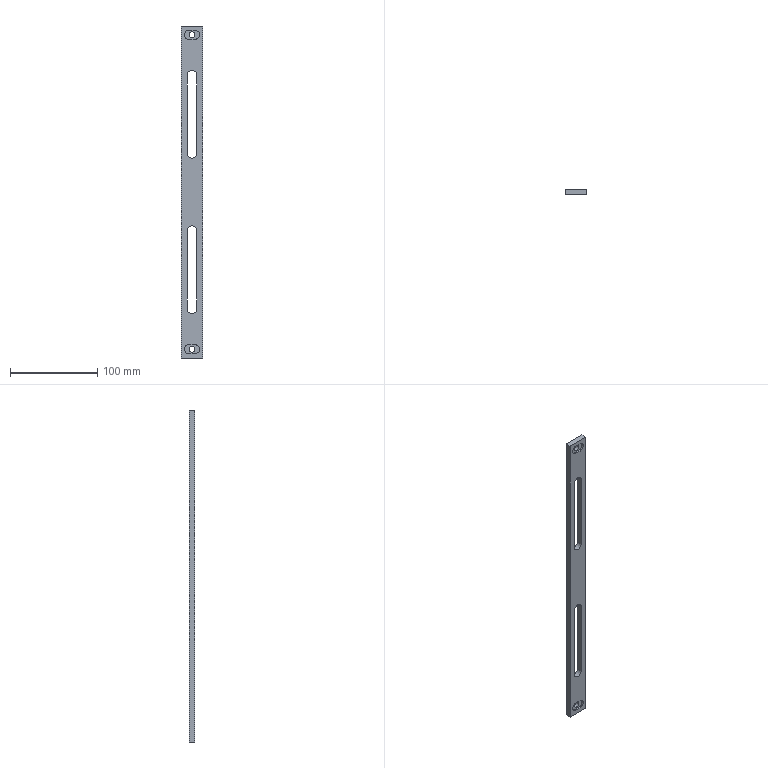Component | SolidWorks | SL021-102-4098.SL4PRT-6 | 1 solid | 30 faces | box 25 x 6 x 380 mm | volume 43743 mm3 | plane 16 | cylinder 14 | commonest cylinder face diameters 10.2 x6 6.5 x4 10.5 x4 | material AL6061
build123d program:
from build123d import *

# Parameters (mm, degrees)
SKETCH1_W                  = 380
SKETCH1_H                  = 25
BOSS_EXTRUDE1_DEPTH        = 3
CUT_EXTRUDE1_DEPTH         = 191.505
F_8_5_8_5_DIAMETER_HOLE1_D = 6.5
CUT_EXTRUDE2_DEPTH         = 2


with BuildPart() as part:
    # Sketch1 → Boss-Extrude1 (new, symmetric)
    with BuildSketch(Plane(origin=(0, 0, 0), x_dir=(1, 0, 0), z_dir=(0, 1, 0))):
        Rectangle(SKETCH1_W, SKETCH1_H)
    extrude(amount=BOSS_EXTRUDE1_DEPTH, both=True)

    # Sketch2 → Cut-Extrude1 (cut, through all)
    with BuildSketch(Plane(origin=(0, 3, 0), x_dir=(1, 0, 0), z_dir=(0, 1, 0))):
        with BuildLine():
            Line((-44, -5.25), (-134, -5.25))
            ThreePointArc((-134, -5.25), (-139.25, 0), (-134, 5.25))
            Line((-134, 5.25), (-44, 5.25))
            ThreePointArc((-44, 5.25), (-38.75, 0), (-44, -5.25))
        make_face()
        with BuildLine():
            Line((44, -5.25), (134, -5.25))
            ThreePointArc((134, -5.25), (139.25, 0), (134, 5.25))
            Line((134, 5.25), (44, 5.25))
            ThreePointArc((44, 5.25), (38.75, 0), (44, -5.25))
        make_face()
    extrude(amount=-CUT_EXTRUDE1_DEPTH, mode=Mode.SUBTRACT)

    # 8.5 _8.5_ Diameter Hole1 (through all)
    with Locations(Plane(origin=(0, -3, 0), x_dir=(-1, 0, 0), z_dir=(0, -1, 0))):
        with Locations((180, 0), (-180, 0)):
            Hole(F_8_5_8_5_DIAMETER_HOLE1_D / 2)

    # Sketch6 → Cut-Extrude2 (cut)
    with BuildSketch(Plane.XZ.offset(3)):
        with BuildLine():
            Line((-174.9, 3.5), (-174.9, -3.5))
            ThreePointArc((-174.9, -3.5), (-180, -8.6), (-185.1, -3.5))
            Line((-185.1, -3.5), (-185.1, 3.5))
            ThreePointArc((-185.1, 3.5), (-180, 8.6), (-174.9, 3.5))
        make_face()
        with BuildLine():
            Line((174.9, 3.5), (174.9, -3.5))
            ThreePointArc((174.9, -3.5), (180, -8.6), (185.1, -3.5))
            Line((185.1, -3.5), (185.1, 3.5))
            ThreePointArc((185.1, 3.5), (180, 8.6), (174.9, 3.5))
        make_face()
    extrude(amount=-CUT_EXTRUDE2_DEPTH, mode=Mode.SUBTRACT)


solid = part.part

# Placed as in the assembly
solid = solid.moved(Location((-48.663, -105.499, -151.378), (0, 90, 0)))
STEP:
#1=COLOUR_RGB('',0.7922,0.8196,0.9333);
#2=FILL_AREA_STYLE_COLOUR('',#1);
#3=FILL_AREA_STYLE('',(#2));
#4=SURFACE_STYLE_FILL_AREA(#3);
#5=SURFACE_SIDE_STYLE('',(#4));
#6=SURFACE_STYLE_USAGE(.BOTH.,#5);
#7=PRESENTATION_STYLE_ASSIGNMENT((#6));
#8=CARTESIAN_POINT('',(-1.577,-4.193,1.127));
#9=VERTEX_POINT('',#8);
#10=CARTESIAN_POINT('',(-1.778,-4.193,1.328));
#11=VERTEX_POINT('',#10);
#12=CARTESIAN_POINT('',(-1.778,-4.193,1.127));
#13=DIRECTION('',(0.,-1.,0.));
#14=DIRECTION('',(-1.,0.,0.));
#15=AXIS2_PLACEMENT_3D('',#12,#13,#14);
#16=CIRCLE('',#15,0.2008);
#17=EDGE_CURVE('',#9,#11,#16,.T.);
#18=ORIENTED_EDGE('',*,*,#17,.F.);
#19=CARTESIAN_POINT('',(-1.577,-4.272,1.127));
#20=VERTEX_POINT('',#19);
#21=CARTESIAN_POINT('',(-1.577,-4.193,1.127));
#22=DIRECTION('',(0.,-1.,0.));
#23=VECTOR('',#22,39.37);
#24=LINE('',#21,#23);
#25=EDGE_CURVE('',#9,#20,#24,.T.);
#26=ORIENTED_EDGE('',*,*,#25,.T.);
#27=CARTESIAN_POINT('',(-1.778,-4.272,1.328));
#28=VERTEX_POINT('',#27);
#29=CARTESIAN_POINT('',(-1.778,-4.272,1.127));
#30=DIRECTION('',(0.,-1.,0.));
#31=DIRECTION('',(-1.,0.,0.));
#32=AXIS2_PLACEMENT_3D('',#29,#30,#31);
#33=CIRCLE('',#32,0.2008);
#34=EDGE_CURVE('',#20,#28,#33,.T.);
#35=ORIENTED_EDGE('',*,*,#34,.T.);
#36=CARTESIAN_POINT('',(-1.778,-4.193,1.328));
#37=DIRECTION('',(0.,-1.,0.));
#38=VECTOR('',#37,39.37);
#39=LINE('',#36,#38);
#40=EDGE_CURVE('',#11,#28,#39,.T.);
#41=ORIENTED_EDGE('',*,*,#40,.F.);
#42=EDGE_LOOP('',(#18,#26,#35,#41));
#43=FACE_OUTER_BOUND('',#42,.T.);
#44=CARTESIAN_POINT('',(-1.778,-4.193,1.127));
#45=DIRECTION('',(0.,-1.,0.));
#46=DIRECTION('',(1.,0.,0.));
#47=AXIS2_PLACEMENT_3D('',#44,#45,#46);
#48=CYLINDRICAL_SURFACE('',#47,0.2008);
#49=ADVANCED_FACE('',(#43),#48,.F.);
#50=CARTESIAN_POINT('',(-1.577,-4.193,-13.046));
#51=VERTEX_POINT('',#50);
#52=CARTESIAN_POINT('',(-1.778,-4.193,-12.846));
#53=VERTEX_POINT('',#52);
#54=CARTESIAN_POINT('',(-1.778,-4.193,-13.046));
#55=DIRECTION('',(0.,-1.,0.));
#56=DIRECTION('',(1.,0.,0.));
#57=AXIS2_PLACEMENT_3D('',#54,#55,#56);
#58=CIRCLE('',#57,0.2008);
#59=EDGE_CURVE('',#51,#53,#58,.T.);
#60=ORIENTED_EDGE('',*,*,#59,.F.);
#61=CARTESIAN_POINT('',(-1.577,-4.272,-13.046));
#62=VERTEX_POINT('',#61);
#63=CARTESIAN_POINT('',(-1.577,-4.193,-13.046));
#64=DIRECTION('',(0.,-1.,0.));
#65=VECTOR('',#64,39.37);
#66=LINE('',#63,#65);
#67=EDGE_CURVE('',#51,#62,#66,.T.);
#68=ORIENTED_EDGE('',*,*,#67,.T.);
#69=CARTESIAN_POINT('',(-1.778,-4.272,-12.846));
#70=VERTEX_POINT('',#69);
#71=CARTESIAN_POINT('',(-1.778,-4.272,-13.046));
#72=DIRECTION('',(0.,-1.,0.));
#73=DIRECTION('',(1.,0.,0.));
#74=AXIS2_PLACEMENT_3D('',#71,#72,#73);
#75=CIRCLE('',#74,0.2008);
#76=EDGE_CURVE('',#62,#70,#75,.T.);
#77=ORIENTED_EDGE('',*,*,#76,.T.);
#78=CARTESIAN_POINT('',(-1.778,-4.193,-12.846));
#79=DIRECTION('',(0.,-1.,0.));
#80=VECTOR('',#79,39.37);
#81=LINE('',#78,#80);
#82=EDGE_CURVE('',#53,#70,#81,.T.);
#83=ORIENTED_EDGE('',*,*,#82,.F.);
#84=EDGE_LOOP('',(#60,#68,#77,#83));
#85=FACE_OUTER_BOUND('',#84,.T.);
#86=CARTESIAN_POINT('',(-1.778,-4.193,-13.046));
#87=DIRECTION('',(0.,-1.,0.));
#88=DIRECTION('',(1.,0.,0.));
#89=AXIS2_PLACEMENT_3D('',#86,#87,#88);
#90=CYLINDRICAL_SURFACE('',#89,0.2008);
#91=ADVANCED_FACE('',(#85),#90,.F.);
#92=CARTESIAN_POINT('',(-2.044,-4.035,1.127));
#93=VERTEX_POINT('',#92);
#94=CARTESIAN_POINT('',(-1.788,-4.035,1.127));
#95=VERTEX_POINT('',#94);
#96=CARTESIAN_POINT('',(-1.916,-4.035,1.127));
#97=DIRECTION('',(0.,-1.,0.));
#98=DIRECTION('',(1.,0.,0.));
#99=AXIS2_PLACEMENT_3D('',#96,#97,#98);
#100=CIRCLE('',#99,0.128);
#101=EDGE_CURVE('',#93,#95,#100,.T.);
#102=ORIENTED_EDGE('',*,*,#101,.F.);
#103=CARTESIAN_POINT('',(-2.044,-4.193,1.127));
#104=VERTEX_POINT('',#103);
#105=CARTESIAN_POINT('',(-2.044,-4.272,1.127));
#106=DIRECTION('',(0.,-1.,0.));
#107=VECTOR('',#106,39.37);
#108=LINE('',#105,#107);
#109=EDGE_CURVE('',#93,#104,#108,.T.);
#110=ORIENTED_EDGE('',*,*,#109,.T.);
#111=CARTESIAN_POINT('',(-1.788,-4.193,1.127));
#112=VERTEX_POINT('',#111);
#113=CARTESIAN_POINT('',(-1.916,-4.193,1.127));
#114=DIRECTION('',(0.,-1.,0.));
#115=DIRECTION('',(-1.,0.,0.));
#116=AXIS2_PLACEMENT_3D('',#113,#114,#115);
#117=CIRCLE('',#116,0.128);
#118=EDGE_CURVE('',#104,#112,#117,.T.);
#119=ORIENTED_EDGE('',*,*,#118,.T.);
#120=CARTESIAN_POINT('',(-1.788,-4.272,1.127));
#121=DIRECTION('',(0.,-1.,0.));
#122=VECTOR('',#121,39.37);
#123=LINE('',#120,#122);
#124=EDGE_CURVE('',#95,#112,#123,.T.);
#125=ORIENTED_EDGE('',*,*,#124,.F.);
#126=EDGE_LOOP('',(#102,#110,#119,#125));
#127=FACE_OUTER_BOUND('',#126,.T.);
#128=CARTESIAN_POINT('',(-1.916,-4.272,1.127));
#129=DIRECTION('',(0.,-1.,0.));
#130=DIRECTION('',(1.,0.,0.));
#131=AXIS2_PLACEMENT_3D('',#128,#129,#130);
#132=CYLINDRICAL_SURFACE('',#131,0.128);
#133=ADVANCED_FACE('',(#127),#132,.F.);
#134=CARTESIAN_POINT('',(-2.044,-4.035,-13.046));
#135=VERTEX_POINT('',#134);
#136=CARTESIAN_POINT('',(-1.788,-4.035,-13.046));
#137=VERTEX_POINT('',#136);
#138=CARTESIAN_POINT('',(-1.916,-4.035,-13.046));
#139=DIRECTION('',(0.,-1.,0.));
#140=DIRECTION('',(1.,0.,0.));
#141=AXIS2_PLACEMENT_3D('',#138,#139,#140);
#142=CIRCLE('',#141,0.128);
#143=EDGE_CURVE('',#135,#137,#142,.T.);
#144=ORIENTED_EDGE('',*,*,#143,.F.);
#145=CARTESIAN_POINT('',(-2.044,-4.193,-13.046));
#146=VERTEX_POINT('',#145);
#147=CARTESIAN_POINT('',(-2.044,-4.272,-13.046));
#148=DIRECTION('',(0.,-1.,0.));
#149=VECTOR('',#148,39.37);
#150=LINE('',#147,#149);
#151=EDGE_CURVE('',#135,#146,#150,.T.);
#152=ORIENTED_EDGE('',*,*,#151,.T.);
#153=CARTESIAN_POINT('',(-1.788,-4.193,-13.046));
#154=VERTEX_POINT('',#153);
#155=CARTESIAN_POINT('',(-1.916,-4.193,-13.046));
#156=DIRECTION('',(-0.,1.,-0.));
#157=DIRECTION('',(1.,0.,0.));
#158=AXIS2_PLACEMENT_3D('',#155,#156,#157);
#159=CIRCLE('',#158,0.128);
#160=EDGE_CURVE('',#154,#146,#159,.T.);
#161=ORIENTED_EDGE('',*,*,#160,.F.);
#162=CARTESIAN_POINT('',(-1.788,-4.272,-13.046));
#163=DIRECTION('',(0.,-1.,0.));
#164=VECTOR('',#163,39.37);
#165=LINE('',#162,#164);
#166=EDGE_CURVE('',#137,#154,#165,.T.);
#167=ORIENTED_EDGE('',*,*,#166,.F.);
#168=EDGE_LOOP('',(#144,#152,#161,#167));
#169=FACE_OUTER_BOUND('',#168,.T.);
#170=CARTESIAN_POINT('',(-1.916,-4.272,-13.046));
#171=DIRECTION('',(0.,-1.,0.));
#172=DIRECTION('',(1.,0.,0.));
#173=AXIS2_PLACEMENT_3D('',#170,#171,#172);
#174=CYLINDRICAL_SURFACE('',#173,0.128);
#175=ADVANCED_FACE('',(#169),#174,.F.);
#176=ORIENTED_EDGE('',*,*,#151,.F.);
#177=CARTESIAN_POINT('',(-1.916,-4.035,-13.046));
#178=DIRECTION('',(0.,-1.,0.));
#179=DIRECTION('',(1.,0.,0.));
#180=AXIS2_PLACEMENT_3D('',#177,#178,#179);
#181=CIRCLE('',#180,0.128);
#182=EDGE_CURVE('',#137,#135,#181,.T.);
#183=ORIENTED_EDGE('',*,*,#182,.F.);
#184=ORIENTED_EDGE('',*,*,#166,.T.);
#185=CARTESIAN_POINT('',(-1.916,-4.193,-13.046));
#186=DIRECTION('',(-0.,1.,-0.));
#187=DIRECTION('',(1.,0.,0.));
#188=AXIS2_PLACEMENT_3D('',#185,#186,#187);
#189=CIRCLE('',#188,0.128);
#190=EDGE_CURVE('',#146,#154,#189,.T.);
#191=ORIENTED_EDGE('',*,*,#190,.F.);
#192=EDGE_LOOP('',(#176,#183,#184,#191));
#193=FACE_OUTER_BOUND('',#192,.T.);
#194=CARTESIAN_POINT('',(-1.916,-4.272,-13.046));
#195=DIRECTION('',(0.,-1.,0.));
#196=DIRECTION('',(1.,0.,0.));
#197=AXIS2_PLACEMENT_3D('',#194,#195,#196);
#198=CYLINDRICAL_SURFACE('',#197,0.128);
#199=ADVANCED_FACE('',(#193),#198,.F.);
#200=CARTESIAN_POINT('',(-2.408,-4.272,1.521));
#201=VERTEX_POINT('',#200);
#202=CARTESIAN_POINT('',(-1.424,-4.272,1.521));
#203=VERTEX_POINT('',#202);
#204=CARTESIAN_POINT('',(-2.408,-4.272,1.521));
#205=DIRECTION('',(1.,0.,0.));
#206=VECTOR('',#205,39.37);
#207=LINE('',#204,#206);
#208=EDGE_CURVE('',#201,#203,#207,.T.);
#209=ORIENTED_EDGE('',*,*,#208,.T.);
#210=CARTESIAN_POINT('',(-1.424,-4.035,1.521));
#211=VERTEX_POINT('',#210);
#212=CARTESIAN_POINT('',(-1.424,-4.035,1.521));
#213=DIRECTION('',(0.,-1.,0.));
#214=VECTOR('',#213,39.37);
#215=LINE('',#212,#214);
#216=EDGE_CURVE('',#211,#203,#215,.T.);
#217=ORIENTED_EDGE('',*,*,#216,.F.);
#218=CARTESIAN_POINT('',(-2.408,-4.035,1.521));
#219=VERTEX_POINT('',#218);
#220=CARTESIAN_POINT('',(-2.408,-4.035,1.521));
#221=DIRECTION('',(1.,0.,0.));
#222=VECTOR('',#221,39.37);
#223=LINE('',#220,#222);
#224=EDGE_CURVE('',#219,#211,#223,.T.);
#225=ORIENTED_EDGE('',*,*,#224,.F.);
#226=CARTESIAN_POINT('',(-2.408,-4.035,1.521));
#227=DIRECTION('',(0.,-1.,0.));
#228=VECTOR('',#227,39.37);
#229=LINE('',#226,#228);
#230=EDGE_CURVE('',#219,#201,#229,.T.);
#231=ORIENTED_EDGE('',*,*,#230,.T.);
#232=EDGE_LOOP('',(#209,#217,#225,#231));
#233=FACE_OUTER_BOUND('',#232,.T.);
#234=CARTESIAN_POINT('',(-2.408,-4.035,1.521));
#235=DIRECTION('',(0.,-0.,-1.));
#236=DIRECTION('',(-1.,-0.,-0.));
#237=AXIS2_PLACEMENT_3D('',#234,#235,#236);
#238=PLANE('',#237);
#239=ADVANCED_FACE('',(#233),#238,.F.);
#240=CARTESIAN_POINT('',(-1.424,-4.272,-13.44));
#241=VERTEX_POINT('',#240);
#242=CARTESIAN_POINT('',(-1.424,-4.272,-13.44));
#243=DIRECTION('',(0.,-0.,-1.));
#244=VECTOR('',#243,39.37);
#245=LINE('',#242,#244);
#246=EDGE_CURVE('',#203,#241,#245,.T.);
#247=ORIENTED_EDGE('',*,*,#246,.T.);
#248=CARTESIAN_POINT('',(-1.424,-4.035,-13.44));
#249=VERTEX_POINT('',#248);
#250=CARTESIAN_POINT('',(-1.424,-4.035,-13.44));
#251=DIRECTION('',(0.,-1.,0.));
#252=VECTOR('',#251,39.37);
#253=LINE('',#250,#252);
#254=EDGE_CURVE('',#249,#241,#253,.T.);
#255=ORIENTED_EDGE('',*,*,#254,.F.);
#256=CARTESIAN_POINT('',(-1.424,-4.035,-13.44));
#257=DIRECTION('',(0.,-0.,-1.));
#258=VECTOR('',#257,39.37);
#259=LINE('',#256,#258);
#260=EDGE_CURVE('',#211,#249,#259,.T.);
#261=ORIENTED_EDGE('',*,*,#260,.F.);
#262=ORIENTED_EDGE('',*,*,#216,.T.);
#263=EDGE_LOOP('',(#247,#255,#261,#262));
#264=FACE_OUTER_BOUND('',#263,.T.);
#265=CARTESIAN_POINT('',(-1.424,-4.035,-13.44));
#266=DIRECTION('',(-1.,-0.,-0.));
#267=DIRECTION('',(-0.,0.,1.));
#268=AXIS2_PLACEMENT_3D('',#265,#266,#267);
#269=PLANE('',#268);
#270=ADVANCED_FACE('',(#264),#269,.F.);
#271=CARTESIAN_POINT('',(-2.408,-4.272,-13.44));
#272=VERTEX_POINT('',#271);
#273=CARTESIAN_POINT('',(-2.408,-4.272,-13.44));
#274=DIRECTION('',(-1.,-0.,-0.));
#275=VECTOR('',#274,39.37);
#276=LINE('',#273,#275);
#277=EDGE_CURVE('',#241,#272,#276,.T.);
#278=ORIENTED_EDGE('',*,*,#277,.T.);
#279=CARTESIAN_POINT('',(-2.408,-4.035,-13.44));
#280=VERTEX_POINT('',#279);
#281=CARTESIAN_POINT('',(-2.408,-4.035,-13.44));
#282=DIRECTION('',(0.,-1.,0.));
#283=VECTOR('',#282,39.37);
#284=LINE('',#281,#283);
#285=EDGE_CURVE('',#280,#272,#284,.T.);
#286=ORIENTED_EDGE('',*,*,#285,.F.);
#287=CARTESIAN_POINT('',(-2.408,-4.035,-13.44));
#288=DIRECTION('',(-1.,-0.,-0.));
#289=VECTOR('',#288,39.37);
#290=LINE('',#287,#289);
#291=EDGE_CURVE('',#249,#280,#290,.T.);
#292=ORIENTED_EDGE('',*,*,#291,.F.);
#293=ORIENTED_EDGE('',*,*,#254,.T.);
#294=EDGE_LOOP('',(#278,#286,#292,#293));
#295=FACE_OUTER_BOUND('',#294,.T.);
#296=CARTESIAN_POINT('',(-2.408,-4.035,-13.44));
#297=DIRECTION('',(-0.,0.,1.));
#298=DIRECTION('',(1.,0.,0.));
#299=AXIS2_PLACEMENT_3D('',#296,#297,#298);
#300=PLANE('',#299);
#301=ADVANCED_FACE('',(#295),#300,.F.);
#302=CARTESIAN_POINT('',(-2.408,-4.272,-13.44));
#303=DIRECTION('',(-0.,0.,1.));
#304=VECTOR('',#303,39.37);
#305=LINE('',#302,#304);
#306=EDGE_CURVE('',#272,#201,#305,.T.);
#307=ORIENTED_EDGE('',*,*,#306,.T.);
#308=ORIENTED_EDGE('',*,*,#230,.F.);
#309=CARTESIAN_POINT('',(-2.408,-4.035,-13.44));
#310=DIRECTION('',(-0.,0.,1.));
#311=VECTOR('',#310,39.37);
#312=LINE('',#309,#311);
#313=EDGE_CURVE('',#280,#219,#312,.T.);
#314=ORIENTED_EDGE('',*,*,#313,.F.);
#315=ORIENTED_EDGE('',*,*,#285,.T.);
#316=EDGE_LOOP('',(#307,#308,#314,#315));
#317=FACE_OUTER_BOUND('',#316,.T.);
#318=CARTESIAN_POINT('',(-2.408,-4.035,-13.44));
#319=DIRECTION('',(1.,0.,0.));
#320=DIRECTION('',(0.,-0.,-1.));
#321=AXIS2_PLACEMENT_3D('',#318,#319,#320);
#322=PLANE('',#321);
#323=ADVANCED_FACE('',(#317),#322,.F.);
#324=ORIENTED_EDGE('',*,*,#182,.T.);
#325=ORIENTED_EDGE('',*,*,#143,.T.);
#326=EDGE_LOOP('',(#324,#325));
#327=FACE_BOUND('',#326,.T.);
#328=CARTESIAN_POINT('',(-1.916,-4.035,1.127));
#329=DIRECTION('',(0.,-1.,0.));
#330=DIRECTION('',(1.,0.,0.));
#331=AXIS2_PLACEMENT_3D('',#328,#329,#330);
#332=CIRCLE('',#331,0.128);
#333=EDGE_CURVE('',#95,#93,#332,.T.);
#334=ORIENTED_EDGE('',*,*,#333,.T.);
#335=ORIENTED_EDGE('',*,*,#101,.T.);
#336=EDGE_LOOP('',(#334,#335));
#337=FACE_BOUND('',#336,.T.);
#338=CARTESIAN_POINT('',(-2.123,-4.035,-4.227));
#339=VERTEX_POINT('',#338);
#340=CARTESIAN_POINT('',(-2.123,-4.035,-0.6842));
#341=VERTEX_POINT('',#340);
#342=CARTESIAN_POINT('',(-2.123,-4.035,-4.227));
#343=DIRECTION('',(-0.,0.,1.));
#344=VECTOR('',#343,39.37);
#345=LINE('',#342,#344);
#346=EDGE_CURVE('',#339,#341,#345,.T.);
#347=ORIENTED_EDGE('',*,*,#346,.F.);
#348=CARTESIAN_POINT('',(-1.709,-4.035,-4.227));
#349=VERTEX_POINT('',#348);
#350=CARTESIAN_POINT('',(-1.916,-4.035,-4.227));
#351=DIRECTION('',(-0.,1.,-0.));
#352=DIRECTION('',(1.,0.,0.));
#353=AXIS2_PLACEMENT_3D('',#350,#351,#352);
#354=CIRCLE('',#353,0.2067);
#355=EDGE_CURVE('',#349,#339,#354,.T.);
#356=ORIENTED_EDGE('',*,*,#355,.F.);
#357=CARTESIAN_POINT('',(-1.709,-4.035,-0.6842));
#358=VERTEX_POINT('',#357);
#359=CARTESIAN_POINT('',(-1.709,-4.035,-4.227));
#360=DIRECTION('',(0.,-0.,-1.));
#361=VECTOR('',#360,39.37);
#362=LINE('',#359,#361);
#363=EDGE_CURVE('',#358,#349,#362,.T.);
#364=ORIENTED_EDGE('',*,*,#363,.F.);
#365=CARTESIAN_POINT('',(-1.916,-4.035,-0.6842));
#366=DIRECTION('',(-0.,1.,-0.));
#367=DIRECTION('',(1.,0.,0.));
#368=AXIS2_PLACEMENT_3D('',#365,#366,#367);
#369=CIRCLE('',#368,0.2067);
#370=EDGE_CURVE('',#341,#358,#369,.T.);
#371=ORIENTED_EDGE('',*,*,#370,.F.);
#372=EDGE_LOOP('',(#347,#356,#364,#371));
#373=FACE_BOUND('',#372,.T.);
#374=CARTESIAN_POINT('',(-1.709,-4.035,-7.692));
#375=VERTEX_POINT('',#374);
#376=CARTESIAN_POINT('',(-1.709,-4.035,-11.235));
#377=VERTEX_POINT('',#376);
#378=CARTESIAN_POINT('',(-1.709,-4.035,-7.692));
#379=DIRECTION('',(0.,-0.,-1.));
#380=VECTOR('',#379,39.37);
#381=LINE('',#378,#380);
#382=EDGE_CURVE('',#375,#377,#381,.T.);
#383=ORIENTED_EDGE('',*,*,#382,.F.);
#384=CARTESIAN_POINT('',(-2.123,-4.035,-7.692));
#385=VERTEX_POINT('',#384);
#386=CARTESIAN_POINT('',(-1.916,-4.035,-7.692));
#387=DIRECTION('',(-0.,1.,-0.));
#388=DIRECTION('',(-1.,0.,0.));
#389=AXIS2_PLACEMENT_3D('',#386,#387,#388);
#390=CIRCLE('',#389,0.2067);
#391=EDGE_CURVE('',#385,#375,#390,.T.);
#392=ORIENTED_EDGE('',*,*,#391,.F.);
#393=CARTESIAN_POINT('',(-2.123,-4.035,-11.235));
#394=VERTEX_POINT('',#393);
#395=CARTESIAN_POINT('',(-2.123,-4.035,-7.692));
#396=DIRECTION('',(-0.,0.,1.));
#397=VECTOR('',#396,39.37);
#398=LINE('',#395,#397);
#399=EDGE_CURVE('',#394,#385,#398,.T.);
#400=ORIENTED_EDGE('',*,*,#399,.F.);
#401=CARTESIAN_POINT('',(-1.916,-4.035,-11.235));
#402=DIRECTION('',(-0.,1.,-0.));
#403=DIRECTION('',(-1.,0.,0.));
#404=AXIS2_PLACEMENT_3D('',#401,#402,#403);
#405=CIRCLE('',#404,0.2067);
#406=EDGE_CURVE('',#377,#394,#405,.T.);
#407=ORIENTED_EDGE('',*,*,#406,.F.);
#408=EDGE_LOOP('',(#383,#392,#400,#407));
#409=FACE_BOUND('',#408,.T.);
#410=ORIENTED_EDGE('',*,*,#224,.T.);
#411=ORIENTED_EDGE('',*,*,#260,.T.);
#412=ORIENTED_EDGE('',*,*,#291,.T.);
#413=ORIENTED_EDGE('',*,*,#313,.T.);
#414=EDGE_LOOP('',(#410,#411,#412,#413));
#415=FACE_OUTER_BOUND('',#414,.T.);
#416=CARTESIAN_POINT('',(-1.916,-4.035,-5.96));
#417=DIRECTION('',(0.,-1.,0.));
#418=DIRECTION('',(1.,0.,0.));
#419=AXIS2_PLACEMENT_3D('',#416,#417,#418);
#420=PLANE('',#419);
#421=ADVANCED_FACE('',(#327,#337,#373,#409,#415),#420,.F.);
#422=CARTESIAN_POINT('',(-2.054,-4.272,1.328));
#423=VERTEX_POINT('',#422);
#424=CARTESIAN_POINT('',(-2.054,-4.272,0.926));
#425=VERTEX_POINT('',#424);
#426=CARTESIAN_POINT('',(-2.054,-4.272,1.127));
#427=DIRECTION('',(0.,-1.,0.));
#428=DIRECTION('',(-1.,0.,0.));
#429=AXIS2_PLACEMENT_3D('',#426,#427,#428);
#430=CIRCLE('',#429,0.2008);
#431=EDGE_CURVE('',#423,#425,#430,.T.);
#432=ORIENTED_EDGE('',*,*,#431,.F.);
#433=CARTESIAN_POINT('',(-2.054,-4.272,1.328));
#434=DIRECTION('',(-1.,-0.,-0.));
#435=VECTOR('',#434,39.37);
#436=LINE('',#433,#435);
#437=EDGE_CURVE('',#28,#423,#436,.T.);
#438=ORIENTED_EDGE('',*,*,#437,.F.);
#439=ORIENTED_EDGE('',*,*,#34,.F.);
#440=CARTESIAN_POINT('',(-1.778,-4.272,0.926));
#441=VERTEX_POINT('',#440);
#442=CARTESIAN_POINT('',(-1.778,-4.272,1.127));
#443=DIRECTION('',(0.,-1.,0.));
#444=DIRECTION('',(-1.,0.,0.));
#445=AXIS2_PLACEMENT_3D('',#442,#443,#444);
#446=CIRCLE('',#445,0.2008);
#447=EDGE_CURVE('',#441,#20,#446,.T.);
#448=ORIENTED_EDGE('',*,*,#447,.F.);
#449=CARTESIAN_POINT('',(-2.054,-4.272,0.926));
#450=DIRECTION('',(1.,0.,0.));
#451=VECTOR('',#450,39.37);
#452=LINE('',#449,#451);
#453=EDGE_CURVE('',#425,#441,#452,.T.);
#454=ORIENTED_EDGE('',*,*,#453,.F.);
#455=EDGE_LOOP('',(#432,#438,#439,#448,#454));
#456=FACE_BOUND('',#455,.T.);
#457=CARTESIAN_POINT('',(-2.054,-4.272,-12.846));
#458=VERTEX_POINT('',#457);
#459=CARTESIAN_POINT('',(-2.054,-4.272,-13.247));
#460=VERTEX_POINT('',#459);
#461=CARTESIAN_POINT('',(-2.054,-4.272,-13.046));
#462=DIRECTION('',(0.,-1.,0.));
#463=DIRECTION('',(1.,0.,0.));
#464=AXIS2_PLACEMENT_3D('',#461,#462,#463);
#465=CIRCLE('',#464,0.2008);
#466=EDGE_CURVE('',#458,#460,#465,.T.);
#467=ORIENTED_EDGE('',*,*,#466,.F.);
#468=CARTESIAN_POINT('',(-2.054,-4.272,-12.846));
#469=DIRECTION('',(-1.,-0.,-0.));
#470=VECTOR('',#469,39.37);
#471=LINE('',#468,#470);
#472=EDGE_CURVE('',#70,#458,#471,.T.);
#473=ORIENTED_EDGE('',*,*,#472,.F.);
#474=ORIENTED_EDGE('',*,*,#76,.F.);
#475=CARTESIAN_POINT('',(-1.778,-4.272,-13.247));
#476=VERTEX_POINT('',#475);
#477=CARTESIAN_POINT('',(-1.778,-4.272,-13.046));
#478=DIRECTION('',(0.,-1.,0.));
#479=DIRECTION('',(1.,0.,0.));
#480=AXIS2_PLACEMENT_3D('',#477,#478,#479);
#481=CIRCLE('',#480,0.2008);
#482=EDGE_CURVE('',#476,#62,#481,.T.);
#483=ORIENTED_EDGE('',*,*,#482,.F.);
#484=CARTESIAN_POINT('',(-2.054,-4.272,-13.247));
#485=DIRECTION('',(1.,0.,0.));
#486=VECTOR('',#485,39.37);
#487=LINE('',#484,#486);
#488=EDGE_CURVE('',#460,#476,#487,.T.);
#489=ORIENTED_EDGE('',*,*,#488,.F.);
#490=EDGE_LOOP('',(#467,#473,#474,#483,#489));
#491=FACE_BOUND('',#490,.T.);
#492=CARTESIAN_POINT('',(-1.709,-4.272,-4.227));
#493=VERTEX_POINT('',#492);
#494=CARTESIAN_POINT('',(-2.123,-4.272,-4.227));
#495=VERTEX_POINT('',#494);
#496=CARTESIAN_POINT('',(-1.916,-4.272,-4.227));
#497=DIRECTION('',(-0.,1.,-0.));
#498=DIRECTION('',(1.,0.,0.));
#499=AXIS2_PLACEMENT_3D('',#496,#497,#498);
#500=CIRCLE('',#499,0.2067);
#501=EDGE_CURVE('',#493,#495,#500,.T.);
#502=ORIENTED_EDGE('',*,*,#501,.T.);
#503=CARTESIAN_POINT('',(-2.123,-4.272,-0.6842));
#504=VERTEX_POINT('',#503);
#505=CARTESIAN_POINT('',(-2.123,-4.272,-4.227));
#506=DIRECTION('',(-0.,0.,1.));
#507=VECTOR('',#506,39.37);
#508=LINE('',#505,#507);
#509=EDGE_CURVE('',#495,#504,#508,.T.);
#510=ORIENTED_EDGE('',*,*,#509,.T.);
#511=CARTESIAN_POINT('',(-1.709,-4.272,-0.6842));
#512=VERTEX_POINT('',#511);
#513=CARTESIAN_POINT('',(-1.916,-4.272,-0.6842));
#514=DIRECTION('',(-0.,1.,-0.));
#515=DIRECTION('',(1.,0.,0.));
#516=AXIS2_PLACEMENT_3D('',#513,#514,#515);
#517=CIRCLE('',#516,0.2067);
#518=EDGE_CURVE('',#504,#512,#517,.T.);
#519=ORIENTED_EDGE('',*,*,#518,.T.);
#520=CARTESIAN_POINT('',(-1.709,-4.272,-4.227));
#521=DIRECTION('',(0.,-0.,-1.));
#522=VECTOR('',#521,39.37);
#523=LINE('',#520,#522);
#524=EDGE_CURVE('',#512,#493,#523,.T.);
#525=ORIENTED_EDGE('',*,*,#524,.T.);
#526=EDGE_LOOP('',(#502,#510,#519,#525));
#527=FACE_BOUND('',#526,.T.);
#528=CARTESIAN_POINT('',(-2.123,-4.272,-7.692));
#529=VERTEX_POINT('',#528);
#530=CARTESIAN_POINT('',(-1.709,-4.272,-7.692));
#531=VERTEX_POINT('',#530);
#532=CARTESIAN_POINT('',(-1.916,-4.272,-7.692));
#533=DIRECTION('',(-0.,1.,-0.));
#534=DIRECTION('',(-1.,0.,0.));
#535=AXIS2_PLACEMENT_3D('',#532,#533,#534);
#536=CIRCLE('',#535,0.2067);
#537=EDGE_CURVE('',#529,#531,#536,.T.);
#538=ORIENTED_EDGE('',*,*,#537,.T.);
#539=CARTESIAN_POINT('',(-1.709,-4.272,-11.235));
#540=VERTEX_POINT('',#539);
#541=CARTESIAN_POINT('',(-1.709,-4.272,-7.692));
#542=DIRECTION('',(0.,-0.,-1.));
#543=VECTOR('',#542,39.37);
#544=LINE('',#541,#543);
#545=EDGE_CURVE('',#531,#540,#544,.T.);
#546=ORIENTED_EDGE('',*,*,#545,.T.);
#547=CARTESIAN_POINT('',(-2.123,-4.272,-11.235));
#548=VERTEX_POINT('',#547);
#549=CARTESIAN_POINT('',(-1.916,-4.272,-11.235));
#550=DIRECTION('',(-0.,1.,-0.));
#551=DIRECTION('',(-1.,0.,0.));
#552=AXIS2_PLACEMENT_3D('',#549,#550,#551);
#553=CIRCLE('',#552,0.2067);
#554=EDGE_CURVE('',#540,#548,#553,.T.);
#555=ORIENTED_EDGE('',*,*,#554,.T.);
#556=CARTESIAN_POINT('',(-2.123,-4.272,-7.692));
#557=DIRECTION('',(-0.,0.,1.));
#558=VECTOR('',#557,39.37);
#559=LINE('',#556,#558);
#560=EDGE_CURVE('',#548,#529,#559,.T.);
#561=ORIENTED_EDGE('',*,*,#560,.T.);
#562=EDGE_LOOP('',(#538,#546,#555,#561));
#563=FACE_BOUND('',#562,.T.);
#564=ORIENTED_EDGE('',*,*,#208,.F.);
#565=ORIENTED_EDGE('',*,*,#306,.F.);
#566=ORIENTED_EDGE('',*,*,#277,.F.);
#567=ORIENTED_EDGE('',*,*,#246,.F.);
#568=EDGE_LOOP('',(#564,#565,#566,#567));
#569=FACE_OUTER_BOUND('',#568,.T.);
#570=CARTESIAN_POINT('',(-1.916,-4.272,-5.96));
#571=DIRECTION('',(0.,-1.,0.));
#572=DIRECTION('',(1.,0.,0.));
#573=AXIS2_PLACEMENT_3D('',#570,#571,#572);
#574=PLANE('',#573);
#575=ADVANCED_FACE('',(#456,#491,#527,#563,#569),#574,.T.);
#576=ORIENTED_EDGE('',*,*,#391,.T.);
#577=CARTESIAN_POINT('',(-1.709,-4.272,-7.692));
#578=DIRECTION('',(-0.,1.,-0.));
#579=VECTOR('',#578,39.37);
#580=LINE('',#577,#579);
#581=EDGE_CURVE('',#531,#375,#580,.T.);
#582=ORIENTED_EDGE('',*,*,#581,.F.);
#583=ORIENTED_EDGE('',*,*,#537,.F.);
#584=CARTESIAN_POINT('',(-2.123,-4.272,-7.692));
#585=DIRECTION('',(-0.,1.,-0.));
#586=VECTOR('',#585,39.37);
#587=LINE('',#584,#586);
#588=EDGE_CURVE('',#529,#385,#587,.T.);
#589=ORIENTED_EDGE('',*,*,#588,.T.);
#590=EDGE_LOOP('',(#576,#582,#583,#589));
#591=FACE_OUTER_BOUND('',#590,.T.);
#592=CARTESIAN_POINT('',(-1.916,-4.272,-7.692));
#593=DIRECTION('',(-0.,1.,-0.));
#594=DIRECTION('',(-1.,0.,0.));
#595=AXIS2_PLACEMENT_3D('',#592,#593,#594);
#596=CYLINDRICAL_SURFACE('',#595,0.2067);
#597=ADVANCED_FACE('',(#591),#596,.F.);
#598=ORIENTED_EDGE('',*,*,#399,.T.);
#599=ORIENTED_EDGE('',*,*,#588,.F.);
#600=ORIENTED_EDGE('',*,*,#560,.F.);
#601=CARTESIAN_POINT('',(-2.123,-4.272,-11.235));
#602=DIRECTION('',(-0.,1.,-0.));
#603=VECTOR('',#602,39.37);
#604=LINE('',#601,#603);
#605=EDGE_CURVE('',#548,#394,#604,.T.);
#606=ORIENTED_EDGE('',*,*,#605,.T.);
#607=EDGE_LOOP('',(#598,#599,#600,#606));
#608=FACE_OUTER_BOUND('',#607,.T.);
#609=CARTESIAN_POINT('',(-2.123,-4.272,-7.692));
#610=DIRECTION('',(-1.,-0.,-0.));
#611=DIRECTION('',(-0.,0.,1.));
#612=AXIS2_PLACEMENT_3D('',#609,#610,#611);
#613=PLANE('',#612);
#614=ADVANCED_FACE('',(#608),#613,.F.);
#615=ORIENTED_EDGE('',*,*,#406,.T.);
#616=ORIENTED_EDGE('',*,*,#605,.F.);
#617=ORIENTED_EDGE('',*,*,#554,.F.);
#618=CARTESIAN_POINT('',(-1.709,-4.272,-11.235));
#619=DIRECTION('',(-0.,1.,-0.));
#620=VECTOR('',#619,39.37);
#621=LINE('',#618,#620);
#622=EDGE_CURVE('',#540,#377,#621,.T.);
#623=ORIENTED_EDGE('',*,*,#622,.T.);
#624=EDGE_LOOP('',(#615,#616,#617,#623));
#625=FACE_OUTER_BOUND('',#624,.T.);
#626=CARTESIAN_POINT('',(-1.916,-4.272,-11.235));
#627=DIRECTION('',(-0.,1.,-0.));
#628=DIRECTION('',(-1.,0.,0.));
#629=AXIS2_PLACEMENT_3D('',#626,#627,#628);
#630=CYLINDRICAL_SURFACE('',#629,0.2067);
#631=ADVANCED_FACE('',(#625),#630,.F.);
#632=ORIENTED_EDGE('',*,*,#382,.T.);
#633=ORIENTED_EDGE('',*,*,#622,.F.);
#634=ORIENTED_EDGE('',*,*,#545,.F.);
#635=ORIENTED_EDGE('',*,*,#581,.T.);
#636=EDGE_LOOP('',(#632,#633,#634,#635));
#637=FACE_OUTER_BOUND('',#636,.T.);
#638=CARTESIAN_POINT('',(-1.709,-4.272,-7.692));
#639=DIRECTION('',(1.,0.,0.));
#640=DIRECTION('',(0.,-0.,-1.));
#641=AXIS2_PLACEMENT_3D('',#638,#639,#640);
#642=PLANE('',#641);
#643=ADVANCED_FACE('',(#637),#642,.F.);
#644=ORIENTED_EDGE('',*,*,#355,.T.);
#645=CARTESIAN_POINT('',(-2.123,-4.272,-4.227));
#646=DIRECTION('',(-0.,1.,-0.));
#647=VECTOR('',#646,39.37);
#648=LINE('',#645,#647);
#649=EDGE_CURVE('',#495,#339,#648,.T.);
#650=ORIENTED_EDGE('',*,*,#649,.F.);
#651=ORIENTED_EDGE('',*,*,#501,.F.);
#652=CARTESIAN_POINT('',(-1.709,-4.272,-4.227));
#653=DIRECTION('',(-0.,1.,-0.));
#654=VECTOR('',#653,39.37);
#655=LINE('',#652,#654);
#656=EDGE_CURVE('',#493,#349,#655,.T.);
#657=ORIENTED_EDGE('',*,*,#656,.T.);
#658=EDGE_LOOP('',(#644,#650,#651,#657));
#659=FACE_OUTER_BOUND('',#658,.T.);
#660=CARTESIAN_POINT('',(-1.916,-4.272,-4.227));
#661=DIRECTION('',(-0.,1.,-0.));
#662=DIRECTION('',(-1.,0.,0.));
#663=AXIS2_PLACEMENT_3D('',#660,#661,#662);
#664=CYLINDRICAL_SURFACE('',#663,0.2067);
#665=ADVANCED_FACE('',(#659),#664,.F.);
#666=ORIENTED_EDGE('',*,*,#363,.T.);
#667=ORIENTED_EDGE('',*,*,#656,.F.);
#668=ORIENTED_EDGE('',*,*,#524,.F.);
#669=CARTESIAN_POINT('',(-1.709,-4.272,-0.6842));
#670=DIRECTION('',(-0.,1.,-0.));
#671=VECTOR('',#670,39.37);
#672=LINE('',#669,#671);
#673=EDGE_CURVE('',#512,#358,#672,.T.);
#674=ORIENTED_EDGE('',*,*,#673,.T.);
#675=EDGE_LOOP('',(#666,#667,#668,#674));
#676=FACE_OUTER_BOUND('',#675,.T.);
#677=CARTESIAN_POINT('',(-1.709,-4.272,-4.227));
#678=DIRECTION('',(1.,0.,0.));
#679=DIRECTION('',(0.,-0.,-1.));
#680=AXIS2_PLACEMENT_3D('',#677,#678,#679);
#681=PLANE('',#680);
#682=ADVANCED_FACE('',(#676),#681,.F.);
#683=ORIENTED_EDGE('',*,*,#370,.T.);
#684=ORIENTED_EDGE('',*,*,#673,.F.);
#685=ORIENTED_EDGE('',*,*,#518,.F.);
#686=CARTESIAN_POINT('',(-2.123,-4.272,-0.6842));
#687=DIRECTION('',(-0.,1.,-0.));
#688=VECTOR('',#687,39.37);
#689=LINE('',#686,#688);
#690=EDGE_CURVE('',#504,#341,#689,.T.);
#691=ORIENTED_EDGE('',*,*,#690,.T.);
#692=EDGE_LOOP('',(#683,#684,#685,#691));
#693=FACE_OUTER_BOUND('',#692,.T.);
#694=CARTESIAN_POINT('',(-1.916,-4.272,-0.6842));
#695=DIRECTION('',(-0.,1.,-0.));
#696=DIRECTION('',(-1.,0.,0.));
#697=AXIS2_PLACEMENT_3D('',#694,#695,#696);
#698=CYLINDRICAL_SURFACE('',#697,0.2067);
#699=ADVANCED_FACE('',(#693),#698,.F.);
#700=ORIENTED_EDGE('',*,*,#346,.T.);
#701=ORIENTED_EDGE('',*,*,#690,.F.);
#702=ORIENTED_EDGE('',*,*,#509,.F.);
#703=ORIENTED_EDGE('',*,*,#649,.T.);
#704=EDGE_LOOP('',(#700,#701,#702,#703));
#705=FACE_OUTER_BOUND('',#704,.T.);
#706=CARTESIAN_POINT('',(-2.123,-4.272,-4.227));
#707=DIRECTION('',(-1.,-0.,-0.));
#708=DIRECTION('',(-0.,0.,1.));
#709=AXIS2_PLACEMENT_3D('',#706,#707,#708);
#710=PLANE('',#709);
#711=ADVANCED_FACE('',(#705),#710,.F.);
#712=ORIENTED_EDGE('',*,*,#109,.F.);
#713=ORIENTED_EDGE('',*,*,#333,.F.);
#714=ORIENTED_EDGE('',*,*,#124,.T.);
#715=CARTESIAN_POINT('',(-1.916,-4.193,1.127));
#716=DIRECTION('',(0.,-1.,0.));
#717=DIRECTION('',(-1.,0.,0.));
#718=AXIS2_PLACEMENT_3D('',#715,#716,#717);
#719=CIRCLE('',#718,0.128);
#720=EDGE_CURVE('',#112,#104,#719,.T.);
#721=ORIENTED_EDGE('',*,*,#720,.T.);
#722=EDGE_LOOP('',(#712,#713,#714,#721));
#723=FACE_OUTER_BOUND('',#722,.T.);
#724=CARTESIAN_POINT('',(-1.916,-4.272,1.127));
#725=DIRECTION('',(0.,-1.,0.));
#726=DIRECTION('',(1.,0.,0.));
#727=AXIS2_PLACEMENT_3D('',#724,#725,#726);
#728=CYLINDRICAL_SURFACE('',#727,0.128);
#729=ADVANCED_FACE('',(#723),#728,.F.);
#730=CARTESIAN_POINT('',(-2.054,-4.193,-12.846));
#731=VERTEX_POINT('',#730);
#732=CARTESIAN_POINT('',(-2.054,-4.193,-13.247));
#733=VERTEX_POINT('',#732);
#734=CARTESIAN_POINT('',(-2.054,-4.193,-13.046));
#735=DIRECTION('',(0.,-1.,0.));
#736=DIRECTION('',(1.,0.,0.));
#737=AXIS2_PLACEMENT_3D('',#734,#735,#736);
#738=CIRCLE('',#737,0.2008);
#739=EDGE_CURVE('',#731,#733,#738,.T.);
#740=ORIENTED_EDGE('',*,*,#739,.T.);
#741=CARTESIAN_POINT('',(-1.778,-4.193,-13.247));
#742=VERTEX_POINT('',#741);
#743=CARTESIAN_POINT('',(-2.054,-4.193,-13.247));
#744=DIRECTION('',(1.,0.,0.));
#745=VECTOR('',#744,39.37);
#746=LINE('',#743,#745);
#747=EDGE_CURVE('',#733,#742,#746,.T.);
#748=ORIENTED_EDGE('',*,*,#747,.T.);
#749=CARTESIAN_POINT('',(-1.778,-4.193,-13.046));
#750=DIRECTION('',(0.,-1.,0.));
#751=DIRECTION('',(1.,0.,0.));
#752=AXIS2_PLACEMENT_3D('',#749,#750,#751);
#753=CIRCLE('',#752,0.2008);
#754=EDGE_CURVE('',#742,#51,#753,.T.);
#755=ORIENTED_EDGE('',*,*,#754,.T.);
#756=ORIENTED_EDGE('',*,*,#59,.T.);
#757=CARTESIAN_POINT('',(-2.054,-4.193,-12.846));
#758=DIRECTION('',(-1.,-0.,-0.));
#759=VECTOR('',#758,39.37);
#760=LINE('',#757,#759);
#761=EDGE_CURVE('',#53,#731,#760,.T.);
#762=ORIENTED_EDGE('',*,*,#761,.T.);
#763=EDGE_LOOP('',(#740,#748,#755,#756,#762));
#764=FACE_OUTER_BOUND('',#763,.T.);
#765=ORIENTED_EDGE('',*,*,#160,.T.);
#766=ORIENTED_EDGE('',*,*,#190,.T.);
#767=EDGE_LOOP('',(#765,#766));
#768=FACE_BOUND('',#767,.T.);
#769=CARTESIAN_POINT('',(-2.054,-4.193,-13.046));
#770=DIRECTION('',(0.,-1.,0.));
#771=DIRECTION('',(1.,0.,0.));
#772=AXIS2_PLACEMENT_3D('',#769,#770,#771);
#773=PLANE('',#772);
#774=ADVANCED_FACE('',(#764,#768),#773,.T.);
#775=ORIENTED_EDGE('',*,*,#466,.T.);
#776=CARTESIAN_POINT('',(-2.054,-4.193,-13.247));
#777=DIRECTION('',(0.,-1.,0.));
#778=VECTOR('',#777,39.37);
#779=LINE('',#776,#778);
#780=EDGE_CURVE('',#733,#460,#779,.T.);
#781=ORIENTED_EDGE('',*,*,#780,.F.);
#782=ORIENTED_EDGE('',*,*,#739,.F.);
#783=CARTESIAN_POINT('',(-2.054,-4.193,-12.846));
#784=DIRECTION('',(0.,-1.,0.));
#785=VECTOR('',#784,39.37);
#786=LINE('',#783,#785);
#787=EDGE_CURVE('',#731,#458,#786,.T.);
#788=ORIENTED_EDGE('',*,*,#787,.T.);
#789=EDGE_LOOP('',(#775,#781,#782,#788));
#790=FACE_OUTER_BOUND('',#789,.T.);
#791=CARTESIAN_POINT('',(-2.054,-4.193,-13.046));
#792=DIRECTION('',(0.,-1.,0.));
#793=DIRECTION('',(1.,0.,0.));
#794=AXIS2_PLACEMENT_3D('',#791,#792,#793);
#795=CYLINDRICAL_SURFACE('',#794,0.2008);
#796=ADVANCED_FACE('',(#790),#795,.F.);
#797=ORIENTED_EDGE('',*,*,#472,.T.);
#798=ORIENTED_EDGE('',*,*,#787,.F.);
#799=ORIENTED_EDGE('',*,*,#761,.F.);
#800=ORIENTED_EDGE('',*,*,#82,.T.);
#801=EDGE_LOOP('',(#797,#798,#799,#800));
#802=FACE_OUTER_BOUND('',#801,.T.);
#803=CARTESIAN_POINT('',(-2.054,-4.193,-12.846));
#804=DIRECTION('',(-0.,0.,1.));
#805=DIRECTION('',(1.,0.,0.));
#806=AXIS2_PLACEMENT_3D('',#803,#804,#805);
#807=PLANE('',#806);
#808=ADVANCED_FACE('',(#802),#807,.F.);
#809=ORIENTED_EDGE('',*,*,#67,.F.);
#810=ORIENTED_EDGE('',*,*,#754,.F.);
#811=CARTESIAN_POINT('',(-1.778,-4.193,-13.247));
#812=DIRECTION('',(0.,-1.,0.));
#813=VECTOR('',#812,39.37);
#814=LINE('',#811,#813);
#815=EDGE_CURVE('',#742,#476,#814,.T.);
#816=ORIENTED_EDGE('',*,*,#815,.T.);
#817=ORIENTED_EDGE('',*,*,#482,.T.);
#818=EDGE_LOOP('',(#809,#810,#816,#817));
#819=FACE_OUTER_BOUND('',#818,.T.);
#820=CARTESIAN_POINT('',(-1.778,-4.193,-13.046));
#821=DIRECTION('',(0.,-1.,0.));
#822=DIRECTION('',(1.,0.,0.));
#823=AXIS2_PLACEMENT_3D('',#820,#821,#822);
#824=CYLINDRICAL_SURFACE('',#823,0.2008);
#825=ADVANCED_FACE('',(#819),#824,.F.);
#826=ORIENTED_EDGE('',*,*,#488,.T.);
#827=ORIENTED_EDGE('',*,*,#815,.F.);
#828=ORIENTED_EDGE('',*,*,#747,.F.);
#829=ORIENTED_EDGE('',*,*,#780,.T.);
#830=EDGE_LOOP('',(#826,#827,#828,#829));
#831=FACE_OUTER_BOUND('',#830,.T.);
#832=CARTESIAN_POINT('',(-2.054,-4.193,-13.247));
#833=DIRECTION('',(0.,-0.,-1.));
#834=DIRECTION('',(-1.,-0.,-0.));
#835=AXIS2_PLACEMENT_3D('',#832,#833,#834);
#836=PLANE('',#835);
#837=ADVANCED_FACE('',(#831),#836,.F.);
#838=CARTESIAN_POINT('',(-2.054,-4.193,1.328));
#839=VERTEX_POINT('',#838);
#840=CARTESIAN_POINT('',(-2.054,-4.193,0.926));
#841=VERTEX_POINT('',#840);
#842=CARTESIAN_POINT('',(-2.054,-4.193,1.127));
#843=DIRECTION('',(0.,-1.,0.));
#844=DIRECTION('',(-1.,0.,0.));
#845=AXIS2_PLACEMENT_3D('',#842,#843,#844);
#846=CIRCLE('',#845,0.2008);
#847=EDGE_CURVE('',#839,#841,#846,.T.);
#848=ORIENTED_EDGE('',*,*,#847,.T.);
#849=CARTESIAN_POINT('',(-1.778,-4.193,0.926));
#850=VERTEX_POINT('',#849);
#851=CARTESIAN_POINT('',(-2.054,-4.193,0.926));
#852=DIRECTION('',(1.,0.,0.));
#853=VECTOR('',#852,39.37);
#854=LINE('',#851,#853);
#855=EDGE_CURVE('',#841,#850,#854,.T.);
#856=ORIENTED_EDGE('',*,*,#855,.T.);
#857=CARTESIAN_POINT('',(-1.778,-4.193,1.127));
#858=DIRECTION('',(0.,-1.,0.));
#859=DIRECTION('',(-1.,0.,0.));
#860=AXIS2_PLACEMENT_3D('',#857,#858,#859);
#861=CIRCLE('',#860,0.2008);
#862=EDGE_CURVE('',#850,#9,#861,.T.);
#863=ORIENTED_EDGE('',*,*,#862,.T.);
#864=ORIENTED_EDGE('',*,*,#17,.T.);
#865=CARTESIAN_POINT('',(-2.054,-4.193,1.328));
#866=DIRECTION('',(-1.,-0.,-0.));
#867=VECTOR('',#866,39.37);
#868=LINE('',#865,#867);
#869=EDGE_CURVE('',#11,#839,#868,.T.);
#870=ORIENTED_EDGE('',*,*,#869,.T.);
#871=EDGE_LOOP('',(#848,#856,#863,#864,#870));
#872=FACE_OUTER_BOUND('',#871,.T.);
#873=ORIENTED_EDGE('',*,*,#720,.F.);
#874=ORIENTED_EDGE('',*,*,#118,.F.);
#875=EDGE_LOOP('',(#873,#874));
#876=FACE_BOUND('',#875,.T.);
#877=CARTESIAN_POINT('',(-2.054,-4.193,1.127));
#878=DIRECTION('',(-0.,1.,-0.));
#879=DIRECTION('',(-1.,-0.,-0.));
#880=AXIS2_PLACEMENT_3D('',#877,#878,#879);
#881=PLANE('',#880);
#882=ADVANCED_FACE('',(#872,#876),#881,.F.);
#883=ORIENTED_EDGE('',*,*,#431,.T.);
#884=CARTESIAN_POINT('',(-2.054,-4.193,0.926));
#885=DIRECTION('',(0.,-1.,0.));
#886=VECTOR('',#885,39.37);
#887=LINE('',#884,#886);
#888=EDGE_CURVE('',#841,#425,#887,.T.);
#889=ORIENTED_EDGE('',*,*,#888,.F.);
#890=ORIENTED_EDGE('',*,*,#847,.F.);
#891=CARTESIAN_POINT('',(-2.054,-4.193,1.328));
#892=DIRECTION('',(0.,-1.,0.));
#893=VECTOR('',#892,39.37);
#894=LINE('',#891,#893);
#895=EDGE_CURVE('',#839,#423,#894,.T.);
#896=ORIENTED_EDGE('',*,*,#895,.T.);
#897=EDGE_LOOP('',(#883,#889,#890,#896));
#898=FACE_OUTER_BOUND('',#897,.T.);
#899=CARTESIAN_POINT('',(-2.054,-4.193,1.127));
#900=DIRECTION('',(0.,-1.,0.));
#901=DIRECTION('',(1.,0.,0.));
#902=AXIS2_PLACEMENT_3D('',#899,#900,#901);
#903=CYLINDRICAL_SURFACE('',#902,0.2008);
#904=ADVANCED_FACE('',(#898),#903,.F.);
#905=ORIENTED_EDGE('',*,*,#437,.T.);
#906=ORIENTED_EDGE('',*,*,#895,.F.);
#907=ORIENTED_EDGE('',*,*,#869,.F.);
#908=ORIENTED_EDGE('',*,*,#40,.T.);
#909=EDGE_LOOP('',(#905,#906,#907,#908));
#910=FACE_OUTER_BOUND('',#909,.T.);
#911=CARTESIAN_POINT('',(-2.054,-4.193,1.328));
#912=DIRECTION('',(-0.,0.,1.));
#913=DIRECTION('',(1.,0.,0.));
#914=AXIS2_PLACEMENT_3D('',#911,#912,#913);
#915=PLANE('',#914);
#916=ADVANCED_FACE('',(#910),#915,.F.);
#917=ORIENTED_EDGE('',*,*,#25,.F.);
#918=ORIENTED_EDGE('',*,*,#862,.F.);
#919=CARTESIAN_POINT('',(-1.778,-4.193,0.926));
#920=DIRECTION('',(0.,-1.,0.));
#921=VECTOR('',#920,39.37);
#922=LINE('',#919,#921);
#923=EDGE_CURVE('',#850,#441,#922,.T.);
#924=ORIENTED_EDGE('',*,*,#923,.T.);
#925=ORIENTED_EDGE('',*,*,#447,.T.);
#926=EDGE_LOOP('',(#917,#918,#924,#925));
#927=FACE_OUTER_BOUND('',#926,.T.);
#928=CARTESIAN_POINT('',(-1.778,-4.193,1.127));
#929=DIRECTION('',(0.,-1.,0.));
#930=DIRECTION('',(1.,0.,0.));
#931=AXIS2_PLACEMENT_3D('',#928,#929,#930);
#932=CYLINDRICAL_SURFACE('',#931,0.2008);
#933=ADVANCED_FACE('',(#927),#932,.F.);
#934=ORIENTED_EDGE('',*,*,#453,.T.);
#935=ORIENTED_EDGE('',*,*,#923,.F.);
#936=ORIENTED_EDGE('',*,*,#855,.F.);
#937=ORIENTED_EDGE('',*,*,#888,.T.);
#938=EDGE_LOOP('',(#934,#935,#936,#937));
#939=FACE_OUTER_BOUND('',#938,.T.);
#940=CARTESIAN_POINT('',(-2.054,-4.193,0.926));
#941=DIRECTION('',(0.,-0.,-1.));
#942=DIRECTION('',(-1.,-0.,-0.));
#943=AXIS2_PLACEMENT_3D('',#940,#941,#942);
#944=PLANE('',#943);
#945=ADVANCED_FACE('',(#939),#944,.F.);
#946=CLOSED_SHELL('',(#49,#91,#133,#175,#199,#239,#270,#301,#323,#421,#575,#597,#614,#631,#643,#665,#682,#699,#711,#729,#774,#796,#808,#825,#837,#882,#904,#916,#933,#945));
#947=MANIFOLD_SOLID_BREP('',#946);
#948=STYLED_ITEM('',(#7),#947);
#949=(LENGTH_UNIT()NAMED_UNIT(*)SI_UNIT($,.METRE.));
#950=LENGTH_MEASURE_WITH_UNIT(LENGTH_MEASURE(0.0254),#949);
#951=DIMENSIONAL_EXPONENTS(1.,0.,0.,0.,0.,0.,0.);
#952=(CONVERSION_BASED_UNIT('',#950)LENGTH_UNIT()NAMED_UNIT(#951));
#953=UNCERTAINTY_MEASURE_WITH_UNIT(LENGTH_MEASURE(0.00001),#952,'','');
#954=(NAMED_UNIT(*)PLANE_ANGLE_UNIT()SI_UNIT($,.RADIAN.));
#955=(NAMED_UNIT(*)SI_UNIT($,.STERADIAN.)SOLID_ANGLE_UNIT());
#956=(GEOMETRIC_REPRESENTATION_CONTEXT(3)GLOBAL_UNCERTAINTY_ASSIGNED_CONTEXT((#953))GLOBAL_UNIT_ASSIGNED_CONTEXT((#952,#954,#955))REPRESENTATION_CONTEXT('',''));
#957=MECHANICAL_DESIGN_GEOMETRIC_PRESENTATION_REPRESENTATION('',(#948),#956);
#958=PRESENTATION_LAYER_ASSIGNMENT('','',(#948));
#959=CARTESIAN_POINT('',(0.,0.,0.));
#960=DIRECTION('',(0.,0.,1.));
#961=DIRECTION('',(1.,0.,0.));
#962=AXIS2_PLACEMENT_3D('',#959,#960,#961);
#963=(LENGTH_UNIT()NAMED_UNIT(*)SI_UNIT($,.METRE.));
#964=LENGTH_MEASURE_WITH_UNIT(LENGTH_MEASURE(0.0254),#963);
#965=DIMENSIONAL_EXPONENTS(1.,0.,0.,0.,0.,0.,0.);
#966=(CONVERSION_BASED_UNIT('',#964)LENGTH_UNIT()NAMED_UNIT(#965));
#967=UNCERTAINTY_MEASURE_WITH_UNIT(LENGTH_MEASURE(0.00001),#966,'','');
#968=(NAMED_UNIT(*)PLANE_ANGLE_UNIT()SI_UNIT($,.RADIAN.));
#969=(NAMED_UNIT(*)SI_UNIT($,.STERADIAN.)SOLID_ANGLE_UNIT());
#970=(GEOMETRIC_REPRESENTATION_CONTEXT(3)GLOBAL_UNCERTAINTY_ASSIGNED_CONTEXT((#967))GLOBAL_UNIT_ASSIGNED_CONTEXT((#966,#968,#969))REPRESENTATION_CONTEXT('',''));
#971=ADVANCED_BREP_SHAPE_REPRESENTATION('',(#947,#962),#970);